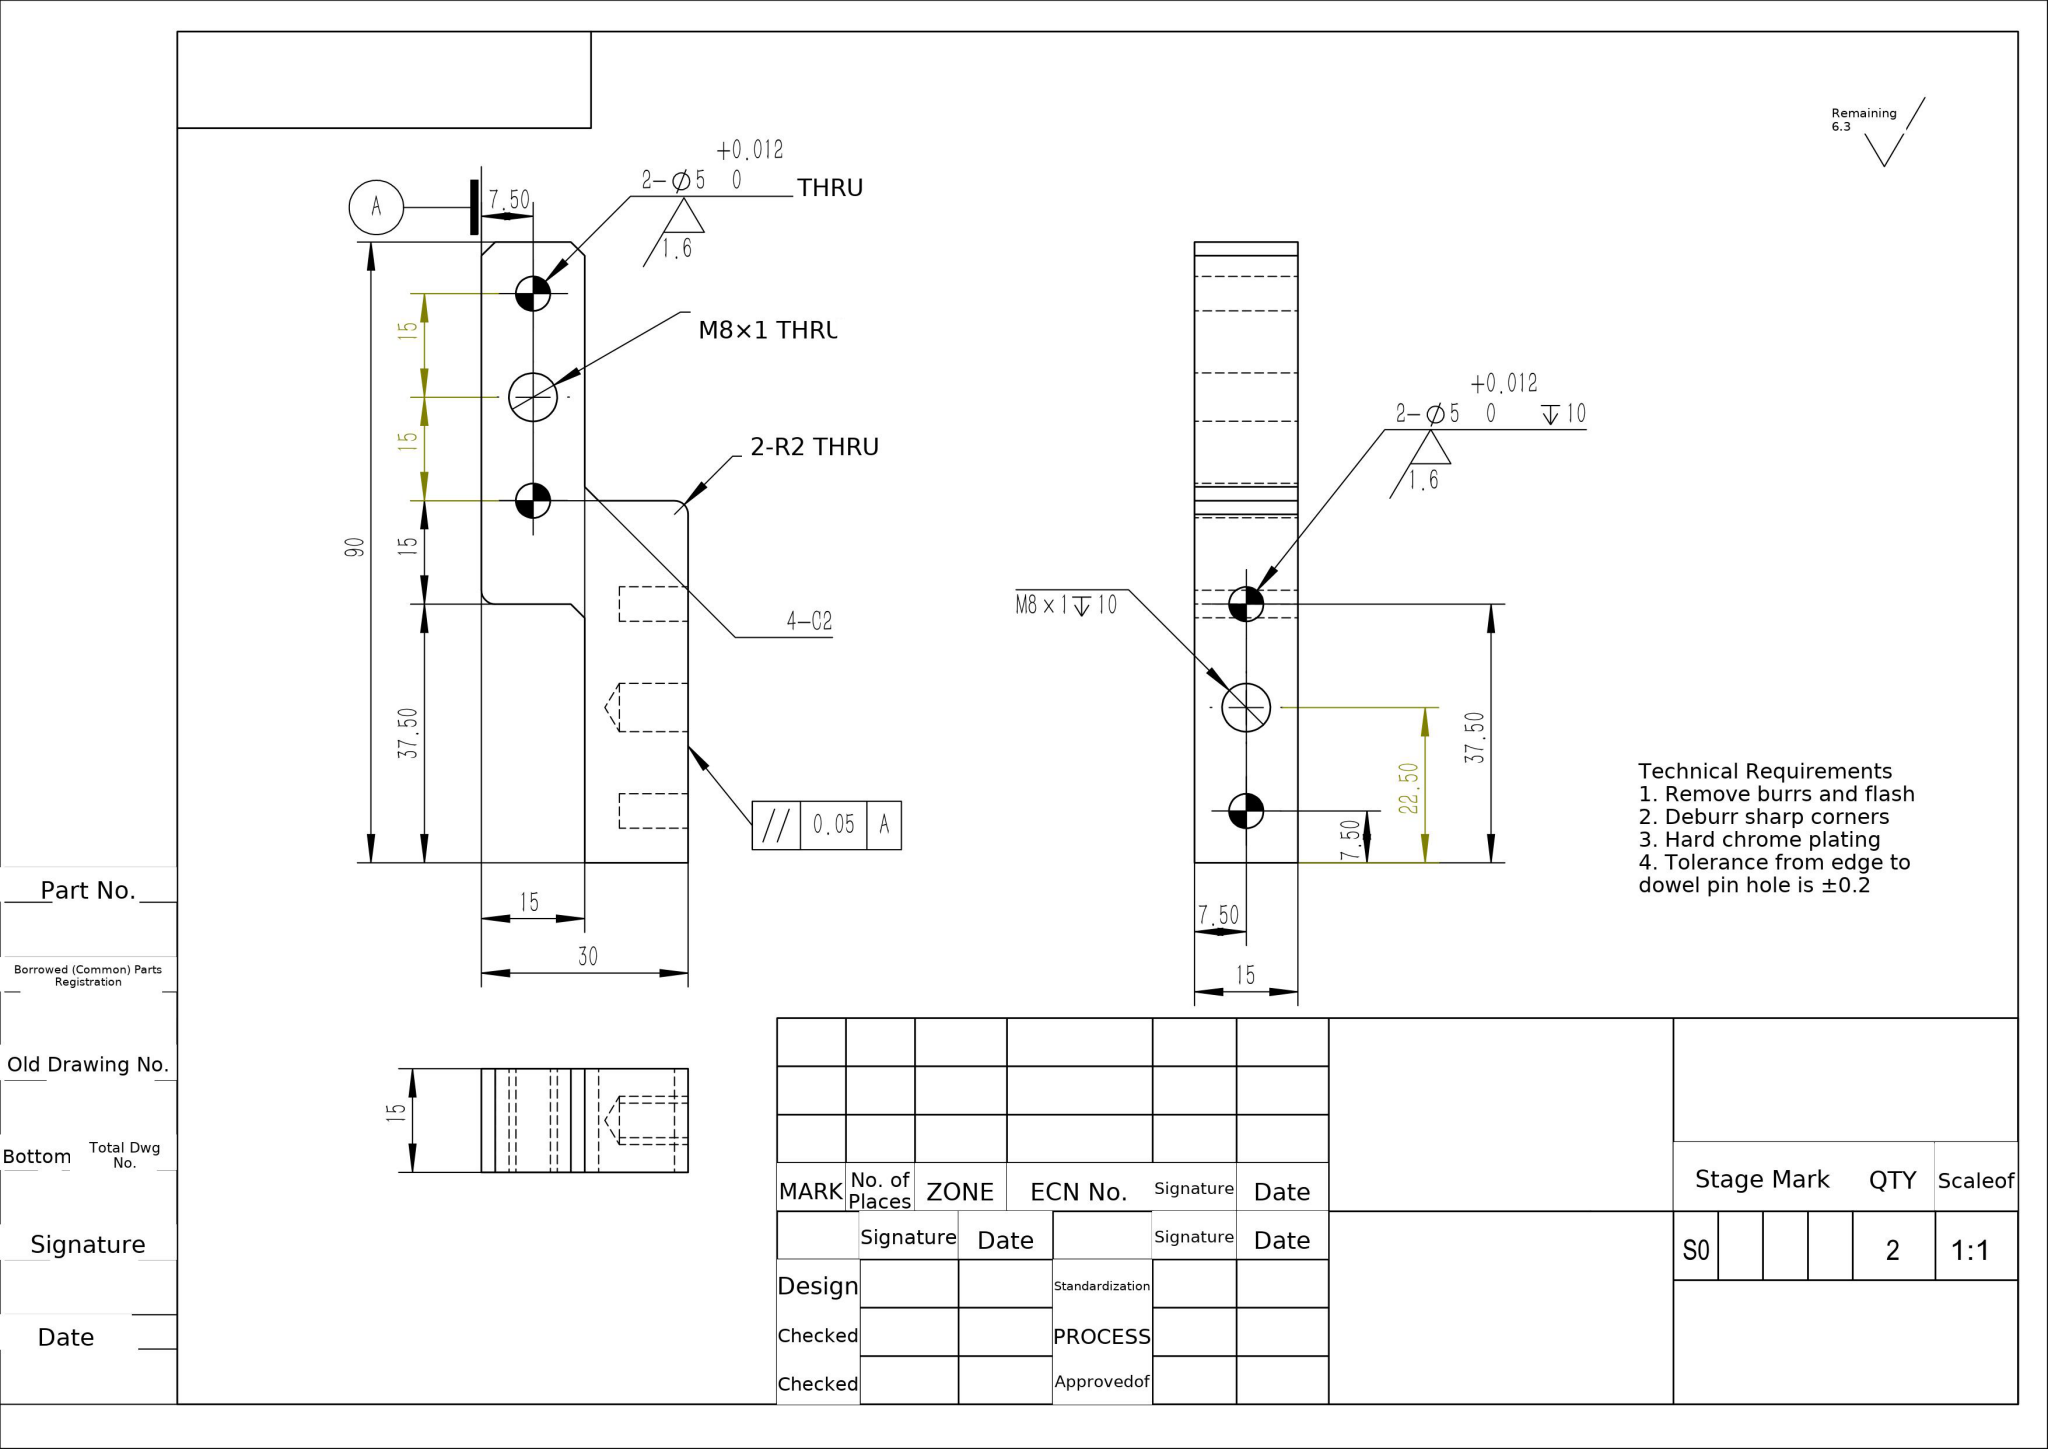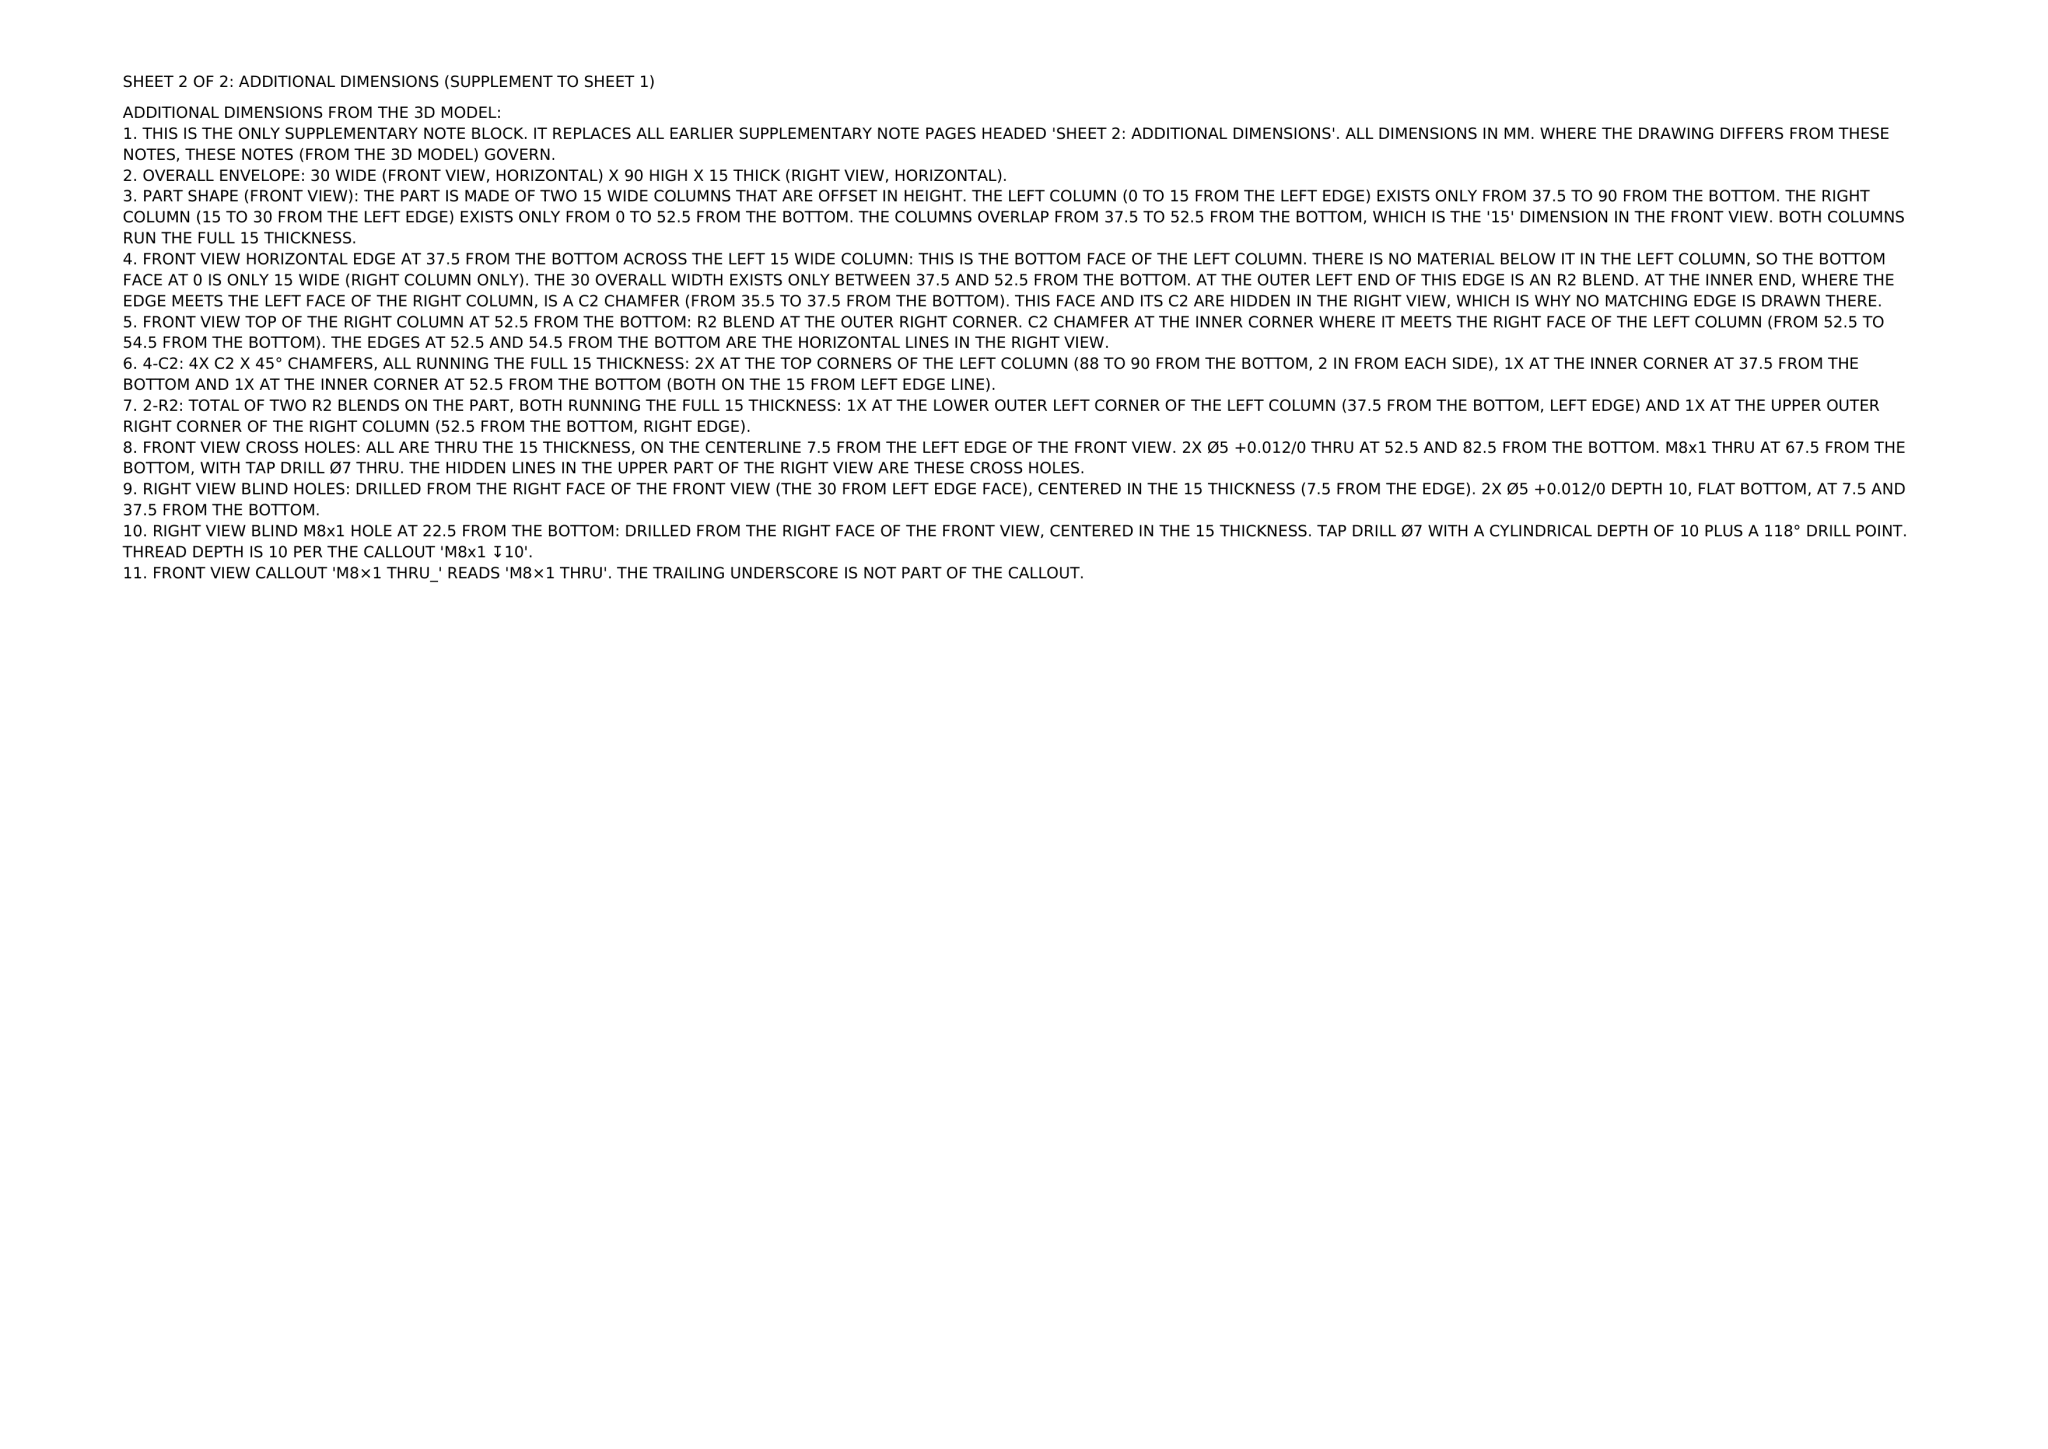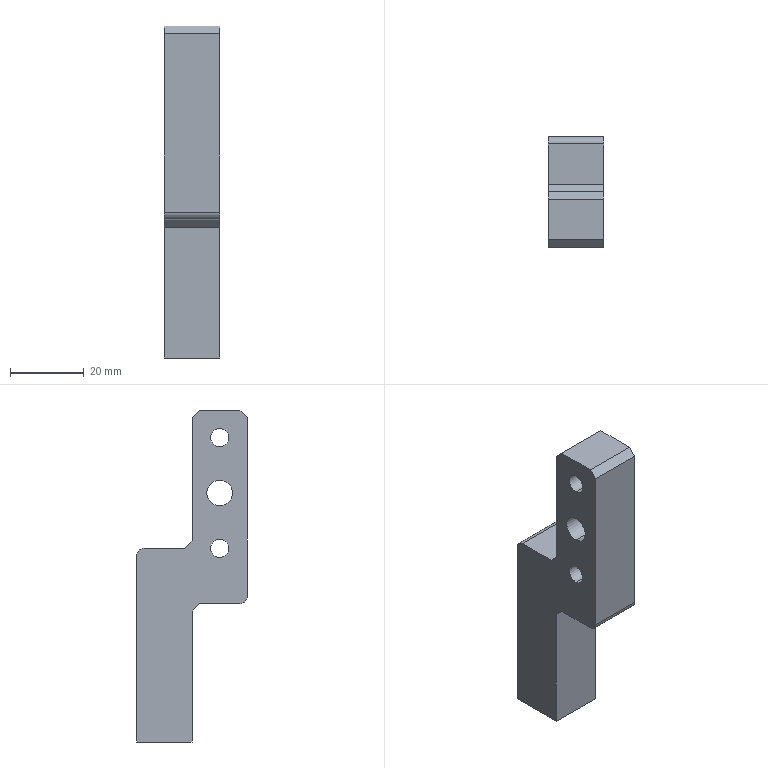Part | NX | mm | 1 solid | 32 faces | box 15 x 30 x 90 mm | volume 21628 mm3 | plane 16 | cylinder 14 | cone 2 | commonest cylinder face diameters 5 x8 7 x4 4 x2